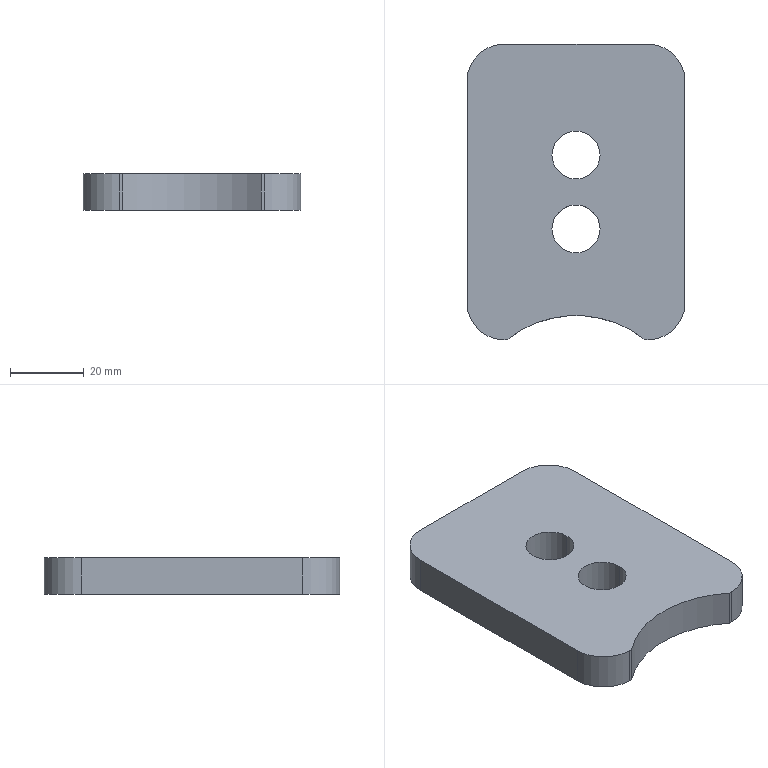Component | SolidWorks | 12ASlidingPlateWheelCover-3 | 1 solid | 16 faces | box 59 x 80 x 10 mm | volume 42016 mm3 | cylinder 9 | plane 7 | commonest cylinder face diameters 13 x4 20 x4 60 x1 | material Q235
build123d program:
from build123d import *

# Parameters (mm, degrees)
SKETCH1_W           = 59
SKETCH1_H           = 80
SKETCH1_R           = 6.5
BOSS_EXTRUDE1_DEPTH = 10
FILLET1_R           = 10
SKETCH2_R           = 30
CUT_EXTRUDE1_DEPTH  = 51.698


with BuildPart() as part:
    # Sketch1 → Boss-Extrude1 (new body)
    with BuildSketch(Plane.XY):
        Rectangle(SKETCH1_W, SKETCH1_H)
        with Locations((0, 10)):
            Circle(SKETCH1_R, mode=Mode.SUBTRACT)
        with Locations((0, -10)):
            Circle(SKETCH1_R, mode=Mode.SUBTRACT)
    extrude(amount=BOSS_EXTRUDE1_DEPTH)

    # Fillet1
    fillet1_edges = [part.edges().sort_by_distance(p)[0] for p in [
        (-29.5, 40, 5),
        (29.5, 40, 5),
        (29.5, -40, 5),
        (-29.5, -40, 5),
    ]]
    fillet(fillet1_edges, radius=FILLET1_R)

    # Sketch2 → Cut-Extrude1 (cut, through all)
    with BuildSketch(Plane.XY.offset(10)):
        with Locations((0, -63.457)):
            Circle(SKETCH2_R)
    extrude(amount=-CUT_EXTRUDE1_DEPTH, mode=Mode.SUBTRACT)


solid = part.part

# Placed as in the assembly
solid = solid.moved(Location((346.598, 136.538, -24.25), (0, 0, 0)))
STEP:
#1=CARTESIAN_POINT('',(13.39,4.982,-0.561));
#2=VERTEX_POINT('',#1);
#3=CARTESIAN_POINT('',(13.902,4.982,-0.561));
#4=VERTEX_POINT('',#3);
#5=CARTESIAN_POINT('',(13.646,4.982,-0.561));
#6=DIRECTION('',(0.,0.,1.));
#7=DIRECTION('',(1.,0.,0.));
#8=AXIS2_PLACEMENT_3D('',#5,#6,#7);
#9=CIRCLE('',#8,0.2559);
#10=EDGE_CURVE('',#2,#4,#9,.T.);
#11=ORIENTED_EDGE('',*,*,#10,.T.);
#12=CARTESIAN_POINT('',(13.902,4.982,-0.9547));
#13=VERTEX_POINT('',#12);
#14=CARTESIAN_POINT('',(13.902,4.982,-0.561));
#15=DIRECTION('',(0.,0.,-1.));
#16=VECTOR('',#15,39.37);
#17=LINE('',#14,#16);
#18=EDGE_CURVE('',#4,#13,#17,.T.);
#19=ORIENTED_EDGE('',*,*,#18,.T.);
#20=CARTESIAN_POINT('',(13.39,4.982,-0.9547));
#21=VERTEX_POINT('',#20);
#22=CARTESIAN_POINT('',(13.646,4.982,-0.9547));
#23=DIRECTION('',(0.,0.,1.));
#24=DIRECTION('',(1.,0.,0.));
#25=AXIS2_PLACEMENT_3D('',#22,#23,#24);
#26=CIRCLE('',#25,0.2559);
#27=EDGE_CURVE('',#21,#13,#26,.T.);
#28=ORIENTED_EDGE('',*,*,#27,.F.);
#29=CARTESIAN_POINT('',(13.39,4.982,-0.561));
#30=DIRECTION('',(0.,0.,-1.));
#31=VECTOR('',#30,39.37);
#32=LINE('',#29,#31);
#33=EDGE_CURVE('',#2,#21,#32,.T.);
#34=ORIENTED_EDGE('',*,*,#33,.F.);
#35=EDGE_LOOP('',(#11,#19,#28,#34));
#36=FACE_OUTER_BOUND('',#35,.T.);
#37=CARTESIAN_POINT('',(13.646,4.982,-0.561));
#38=DIRECTION('',(0.,0.,-1.));
#39=DIRECTION('',(-1.,0.,0.));
#40=AXIS2_PLACEMENT_3D('',#37,#38,#39);
#41=CYLINDRICAL_SURFACE('',#40,0.2559);
#42=ADVANCED_FACE('',(#36),#41,.F.);
#43=CARTESIAN_POINT('',(13.39,5.769,-0.561));
#44=VERTEX_POINT('',#43);
#45=CARTESIAN_POINT('',(13.902,5.769,-0.561));
#46=VERTEX_POINT('',#45);
#47=CARTESIAN_POINT('',(13.646,5.769,-0.561));
#48=DIRECTION('',(0.,0.,1.));
#49=DIRECTION('',(1.,0.,0.));
#50=AXIS2_PLACEMENT_3D('',#47,#48,#49);
#51=CIRCLE('',#50,0.2559);
#52=EDGE_CURVE('',#44,#46,#51,.T.);
#53=ORIENTED_EDGE('',*,*,#52,.T.);
#54=CARTESIAN_POINT('',(13.902,5.769,-0.9547));
#55=VERTEX_POINT('',#54);
#56=CARTESIAN_POINT('',(13.902,5.769,-0.561));
#57=DIRECTION('',(0.,0.,-1.));
#58=VECTOR('',#57,39.37);
#59=LINE('',#56,#58);
#60=EDGE_CURVE('',#46,#55,#59,.T.);
#61=ORIENTED_EDGE('',*,*,#60,.T.);
#62=CARTESIAN_POINT('',(13.39,5.769,-0.9547));
#63=VERTEX_POINT('',#62);
#64=CARTESIAN_POINT('',(13.646,5.769,-0.9547));
#65=DIRECTION('',(0.,0.,1.));
#66=DIRECTION('',(1.,0.,0.));
#67=AXIS2_PLACEMENT_3D('',#64,#65,#66);
#68=CIRCLE('',#67,0.2559);
#69=EDGE_CURVE('',#63,#55,#68,.T.);
#70=ORIENTED_EDGE('',*,*,#69,.F.);
#71=CARTESIAN_POINT('',(13.39,5.769,-0.561));
#72=DIRECTION('',(0.,0.,-1.));
#73=VECTOR('',#72,39.37);
#74=LINE('',#71,#73);
#75=EDGE_CURVE('',#44,#63,#74,.T.);
#76=ORIENTED_EDGE('',*,*,#75,.F.);
#77=EDGE_LOOP('',(#53,#61,#70,#76));
#78=FACE_OUTER_BOUND('',#77,.T.);
#79=CARTESIAN_POINT('',(13.646,5.769,-0.561));
#80=DIRECTION('',(0.,0.,-1.));
#81=DIRECTION('',(-1.,0.,0.));
#82=AXIS2_PLACEMENT_3D('',#79,#80,#81);
#83=CYLINDRICAL_SURFACE('',#82,0.2559);
#84=ADVANCED_FACE('',(#78),#83,.F.);
#85=CARTESIAN_POINT('',(12.878,3.801,-0.9547));
#86=VERTEX_POINT('',#85);
#87=CARTESIAN_POINT('',(12.909,3.801,-0.9547));
#88=VERTEX_POINT('',#87);
#89=CARTESIAN_POINT('',(12.484,3.801,-0.9547));
#90=DIRECTION('',(1.,0.,0.));
#91=VECTOR('',#90,39.37);
#92=LINE('',#89,#91);
#93=EDGE_CURVE('',#86,#88,#92,.T.);
#94=ORIENTED_EDGE('',*,*,#93,.T.);
#95=CARTESIAN_POINT('',(12.909,3.801,-0.561));
#96=VERTEX_POINT('',#95);
#97=CARTESIAN_POINT('',(12.909,3.801,-0.9547));
#98=DIRECTION('',(0.,0.,1.));
#99=VECTOR('',#98,39.37);
#100=LINE('',#97,#99);
#101=EDGE_CURVE('',#88,#96,#100,.T.);
#102=ORIENTED_EDGE('',*,*,#101,.T.);
#103=CARTESIAN_POINT('',(12.878,3.801,-0.561));
#104=VERTEX_POINT('',#103);
#105=CARTESIAN_POINT('',(12.484,3.801,-0.561));
#106=DIRECTION('',(1.,0.,0.));
#107=VECTOR('',#106,39.37);
#108=LINE('',#105,#107);
#109=EDGE_CURVE('',#104,#96,#108,.T.);
#110=ORIENTED_EDGE('',*,*,#109,.F.);
#111=CARTESIAN_POINT('',(12.878,3.801,-0.561));
#112=DIRECTION('',(0.,0.,-1.));
#113=VECTOR('',#112,39.37);
#114=LINE('',#111,#113);
#115=EDGE_CURVE('',#104,#86,#114,.T.);
#116=ORIENTED_EDGE('',*,*,#115,.T.);
#117=EDGE_LOOP('',(#94,#102,#110,#116));
#118=FACE_OUTER_BOUND('',#117,.T.);
#119=CARTESIAN_POINT('',(12.484,3.801,-0.561));
#120=DIRECTION('',(0.,1.,0.));
#121=DIRECTION('',(0.,0.,1.));
#122=AXIS2_PLACEMENT_3D('',#119,#120,#121);
#123=PLANE('',#122);
#124=ADVANCED_FACE('',(#118),#123,.F.);
#125=CARTESIAN_POINT('',(14.382,3.801,-0.561));
#126=VERTEX_POINT('',#125);
#127=CARTESIAN_POINT('',(13.646,2.877,-0.561));
#128=DIRECTION('',(0.,0.,1.));
#129=DIRECTION('',(1.,0.,0.));
#130=AXIS2_PLACEMENT_3D('',#127,#128,#129);
#131=CIRCLE('',#130,1.181);
#132=EDGE_CURVE('',#126,#96,#131,.T.);
#133=ORIENTED_EDGE('',*,*,#132,.F.);
#134=CARTESIAN_POINT('',(14.413,3.801,-0.561));
#135=VERTEX_POINT('',#134);
#136=CARTESIAN_POINT('',(12.484,3.801,-0.561));
#137=DIRECTION('',(1.,0.,0.));
#138=VECTOR('',#137,39.37);
#139=LINE('',#136,#138);
#140=EDGE_CURVE('',#126,#135,#139,.T.);
#141=ORIENTED_EDGE('',*,*,#140,.T.);
#142=CARTESIAN_POINT('',(14.807,4.194,-0.561));
#143=VERTEX_POINT('',#142);
#144=CARTESIAN_POINT('',(14.413,4.194,-0.561));
#145=DIRECTION('',(0.,0.,1.));
#146=DIRECTION('',(1.,0.,0.));
#147=AXIS2_PLACEMENT_3D('',#144,#145,#146);
#148=CIRCLE('',#147,0.3937);
#149=EDGE_CURVE('',#135,#143,#148,.T.);
#150=ORIENTED_EDGE('',*,*,#149,.T.);
#151=CARTESIAN_POINT('',(14.807,6.557,-0.561));
#152=VERTEX_POINT('',#151);
#153=CARTESIAN_POINT('',(14.807,6.95,-0.561));
#154=DIRECTION('',(-0.,1.,0.));
#155=VECTOR('',#154,39.37);
#156=LINE('',#153,#155);
#157=EDGE_CURVE('',#143,#152,#156,.T.);
#158=ORIENTED_EDGE('',*,*,#157,.T.);
#159=CARTESIAN_POINT('',(14.413,6.95,-0.561));
#160=VERTEX_POINT('',#159);
#161=CARTESIAN_POINT('',(14.413,6.557,-0.561));
#162=DIRECTION('',(0.,0.,1.));
#163=DIRECTION('',(1.,0.,0.));
#164=AXIS2_PLACEMENT_3D('',#161,#162,#163);
#165=CIRCLE('',#164,0.3937);
#166=EDGE_CURVE('',#152,#160,#165,.T.);
#167=ORIENTED_EDGE('',*,*,#166,.T.);
#168=CARTESIAN_POINT('',(12.878,6.95,-0.561));
#169=VERTEX_POINT('',#168);
#170=CARTESIAN_POINT('',(12.484,6.95,-0.561));
#171=DIRECTION('',(-1.,-0.,0.));
#172=VECTOR('',#171,39.37);
#173=LINE('',#170,#172);
#174=EDGE_CURVE('',#160,#169,#173,.T.);
#175=ORIENTED_EDGE('',*,*,#174,.T.);
#176=CARTESIAN_POINT('',(12.484,6.557,-0.561));
#177=VERTEX_POINT('',#176);
#178=CARTESIAN_POINT('',(12.878,6.557,-0.561));
#179=DIRECTION('',(0.,0.,1.));
#180=DIRECTION('',(1.,0.,0.));
#181=AXIS2_PLACEMENT_3D('',#178,#179,#180);
#182=CIRCLE('',#181,0.3937);
#183=EDGE_CURVE('',#169,#177,#182,.T.);
#184=ORIENTED_EDGE('',*,*,#183,.T.);
#185=CARTESIAN_POINT('',(12.484,4.194,-0.561));
#186=VERTEX_POINT('',#185);
#187=CARTESIAN_POINT('',(12.484,6.95,-0.561));
#188=DIRECTION('',(0.,-1.,0.));
#189=VECTOR('',#188,39.37);
#190=LINE('',#187,#189);
#191=EDGE_CURVE('',#177,#186,#190,.T.);
#192=ORIENTED_EDGE('',*,*,#191,.T.);
#193=CARTESIAN_POINT('',(12.878,4.194,-0.561));
#194=DIRECTION('',(0.,0.,1.));
#195=DIRECTION('',(1.,0.,0.));
#196=AXIS2_PLACEMENT_3D('',#193,#194,#195);
#197=CIRCLE('',#196,0.3937);
#198=EDGE_CURVE('',#186,#104,#197,.T.);
#199=ORIENTED_EDGE('',*,*,#198,.T.);
#200=ORIENTED_EDGE('',*,*,#109,.T.);
#201=EDGE_LOOP('',(#133,#141,#150,#158,#167,#175,#184,#192,#199,#200));
#202=FACE_OUTER_BOUND('',#201,.T.);
#203=ORIENTED_EDGE('',*,*,#52,.F.);
#204=CARTESIAN_POINT('',(13.646,5.769,-0.561));
#205=DIRECTION('',(0.,0.,1.));
#206=DIRECTION('',(1.,0.,0.));
#207=AXIS2_PLACEMENT_3D('',#204,#205,#206);
#208=CIRCLE('',#207,0.2559);
#209=EDGE_CURVE('',#46,#44,#208,.T.);
#210=ORIENTED_EDGE('',*,*,#209,.F.);
#211=EDGE_LOOP('',(#203,#210));
#212=FACE_BOUND('',#211,.T.);
#213=ORIENTED_EDGE('',*,*,#10,.F.);
#214=CARTESIAN_POINT('',(13.646,4.982,-0.561));
#215=DIRECTION('',(0.,0.,1.));
#216=DIRECTION('',(1.,0.,0.));
#217=AXIS2_PLACEMENT_3D('',#214,#215,#216);
#218=CIRCLE('',#217,0.2559);
#219=EDGE_CURVE('',#4,#2,#218,.T.);
#220=ORIENTED_EDGE('',*,*,#219,.F.);
#221=EDGE_LOOP('',(#213,#220));
#222=FACE_BOUND('',#221,.T.);
#223=CARTESIAN_POINT('',(13.646,5.376,-0.561));
#224=DIRECTION('',(0.,0.,1.));
#225=DIRECTION('',(1.,0.,0.));
#226=AXIS2_PLACEMENT_3D('',#223,#224,#225);
#227=PLANE('',#226);
#228=ADVANCED_FACE('',(#202,#212,#222),#227,.T.);
#229=CARTESIAN_POINT('',(14.382,3.801,-0.9547));
#230=VERTEX_POINT('',#229);
#231=CARTESIAN_POINT('',(14.413,3.801,-0.9547));
#232=VERTEX_POINT('',#231);
#233=CARTESIAN_POINT('',(12.484,3.801,-0.9547));
#234=DIRECTION('',(1.,0.,0.));
#235=VECTOR('',#234,39.37);
#236=LINE('',#233,#235);
#237=EDGE_CURVE('',#230,#232,#236,.T.);
#238=ORIENTED_EDGE('',*,*,#237,.F.);
#239=CARTESIAN_POINT('',(13.646,2.877,-0.9547));
#240=DIRECTION('',(0.,0.,1.));
#241=DIRECTION('',(1.,0.,0.));
#242=AXIS2_PLACEMENT_3D('',#239,#240,#241);
#243=CIRCLE('',#242,1.181);
#244=EDGE_CURVE('',#230,#88,#243,.T.);
#245=ORIENTED_EDGE('',*,*,#244,.T.);
#246=ORIENTED_EDGE('',*,*,#93,.F.);
#247=CARTESIAN_POINT('',(12.484,4.194,-0.9547));
#248=VERTEX_POINT('',#247);
#249=CARTESIAN_POINT('',(12.878,4.194,-0.9547));
#250=DIRECTION('',(0.,0.,-1.));
#251=DIRECTION('',(1.,0.,0.));
#252=AXIS2_PLACEMENT_3D('',#249,#250,#251);
#253=CIRCLE('',#252,0.3937);
#254=EDGE_CURVE('',#86,#248,#253,.T.);
#255=ORIENTED_EDGE('',*,*,#254,.T.);
#256=CARTESIAN_POINT('',(12.484,6.557,-0.9547));
#257=VERTEX_POINT('',#256);
#258=CARTESIAN_POINT('',(12.484,6.95,-0.9547));
#259=DIRECTION('',(0.,-1.,0.));
#260=VECTOR('',#259,39.37);
#261=LINE('',#258,#260);
#262=EDGE_CURVE('',#257,#248,#261,.T.);
#263=ORIENTED_EDGE('',*,*,#262,.F.);
#264=CARTESIAN_POINT('',(12.878,6.95,-0.9547));
#265=VERTEX_POINT('',#264);
#266=CARTESIAN_POINT('',(12.878,6.557,-0.9547));
#267=DIRECTION('',(0.,0.,-1.));
#268=DIRECTION('',(1.,0.,0.));
#269=AXIS2_PLACEMENT_3D('',#266,#267,#268);
#270=CIRCLE('',#269,0.3937);
#271=EDGE_CURVE('',#257,#265,#270,.T.);
#272=ORIENTED_EDGE('',*,*,#271,.T.);
#273=CARTESIAN_POINT('',(14.413,6.95,-0.9547));
#274=VERTEX_POINT('',#273);
#275=CARTESIAN_POINT('',(12.484,6.95,-0.9547));
#276=DIRECTION('',(-1.,-0.,0.));
#277=VECTOR('',#276,39.37);
#278=LINE('',#275,#277);
#279=EDGE_CURVE('',#274,#265,#278,.T.);
#280=ORIENTED_EDGE('',*,*,#279,.F.);
#281=CARTESIAN_POINT('',(14.807,6.557,-0.9547));
#282=VERTEX_POINT('',#281);
#283=CARTESIAN_POINT('',(14.413,6.557,-0.9547));
#284=DIRECTION('',(0.,0.,-1.));
#285=DIRECTION('',(1.,0.,0.));
#286=AXIS2_PLACEMENT_3D('',#283,#284,#285);
#287=CIRCLE('',#286,0.3937);
#288=EDGE_CURVE('',#274,#282,#287,.T.);
#289=ORIENTED_EDGE('',*,*,#288,.T.);
#290=CARTESIAN_POINT('',(14.807,4.194,-0.9547));
#291=VERTEX_POINT('',#290);
#292=CARTESIAN_POINT('',(14.807,6.95,-0.9547));
#293=DIRECTION('',(-0.,1.,0.));
#294=VECTOR('',#293,39.37);
#295=LINE('',#292,#294);
#296=EDGE_CURVE('',#291,#282,#295,.T.);
#297=ORIENTED_EDGE('',*,*,#296,.F.);
#298=CARTESIAN_POINT('',(14.413,4.194,-0.9547));
#299=DIRECTION('',(0.,0.,-1.));
#300=DIRECTION('',(1.,0.,0.));
#301=AXIS2_PLACEMENT_3D('',#298,#299,#300);
#302=CIRCLE('',#301,0.3937);
#303=EDGE_CURVE('',#291,#232,#302,.T.);
#304=ORIENTED_EDGE('',*,*,#303,.T.);
#305=EDGE_LOOP('',(#238,#245,#246,#255,#263,#272,#280,#289,#297,#304));
#306=FACE_OUTER_BOUND('',#305,.T.);
#307=ORIENTED_EDGE('',*,*,#69,.T.);
#308=CARTESIAN_POINT('',(13.646,5.769,-0.9547));
#309=DIRECTION('',(0.,0.,1.));
#310=DIRECTION('',(1.,0.,0.));
#311=AXIS2_PLACEMENT_3D('',#308,#309,#310);
#312=CIRCLE('',#311,0.2559);
#313=EDGE_CURVE('',#55,#63,#312,.T.);
#314=ORIENTED_EDGE('',*,*,#313,.T.);
#315=EDGE_LOOP('',(#307,#314));
#316=FACE_BOUND('',#315,.T.);
#317=ORIENTED_EDGE('',*,*,#27,.T.);
#318=CARTESIAN_POINT('',(13.646,4.982,-0.9547));
#319=DIRECTION('',(0.,0.,1.));
#320=DIRECTION('',(1.,0.,0.));
#321=AXIS2_PLACEMENT_3D('',#318,#319,#320);
#322=CIRCLE('',#321,0.2559);
#323=EDGE_CURVE('',#13,#21,#322,.T.);
#324=ORIENTED_EDGE('',*,*,#323,.T.);
#325=EDGE_LOOP('',(#317,#324));
#326=FACE_BOUND('',#325,.T.);
#327=CARTESIAN_POINT('',(13.646,5.376,-0.9547));
#328=DIRECTION('',(0.,0.,1.));
#329=DIRECTION('',(1.,0.,0.));
#330=AXIS2_PLACEMENT_3D('',#327,#328,#329);
#331=PLANE('',#330);
#332=ADVANCED_FACE('',(#306,#316,#326),#331,.F.);
#333=ORIENTED_EDGE('',*,*,#262,.T.);
#334=CARTESIAN_POINT('',(12.484,4.194,-0.561));
#335=DIRECTION('',(0.,0.,1.));
#336=VECTOR('',#335,39.37);
#337=LINE('',#334,#336);
#338=EDGE_CURVE('',#248,#186,#337,.T.);
#339=ORIENTED_EDGE('',*,*,#338,.T.);
#340=ORIENTED_EDGE('',*,*,#191,.F.);
#341=CARTESIAN_POINT('',(12.484,6.557,-0.561));
#342=DIRECTION('',(0.,0.,-1.));
#343=VECTOR('',#342,39.37);
#344=LINE('',#341,#343);
#345=EDGE_CURVE('',#177,#257,#344,.T.);
#346=ORIENTED_EDGE('',*,*,#345,.T.);
#347=EDGE_LOOP('',(#333,#339,#340,#346));
#348=FACE_OUTER_BOUND('',#347,.T.);
#349=CARTESIAN_POINT('',(12.484,6.95,-0.561));
#350=DIRECTION('',(1.,0.,0.));
#351=DIRECTION('',(-0.,1.,0.));
#352=AXIS2_PLACEMENT_3D('',#349,#350,#351);
#353=PLANE('',#352);
#354=ADVANCED_FACE('',(#348),#353,.F.);
#355=ORIENTED_EDGE('',*,*,#140,.F.);
#356=CARTESIAN_POINT('',(14.382,3.801,-0.9547));
#357=DIRECTION('',(0.,0.,-1.));
#358=VECTOR('',#357,39.37);
#359=LINE('',#356,#358);
#360=EDGE_CURVE('',#126,#230,#359,.T.);
#361=ORIENTED_EDGE('',*,*,#360,.T.);
#362=ORIENTED_EDGE('',*,*,#237,.T.);
#363=CARTESIAN_POINT('',(14.413,3.801,-0.561));
#364=DIRECTION('',(0.,0.,1.));
#365=VECTOR('',#364,39.37);
#366=LINE('',#363,#365);
#367=EDGE_CURVE('',#232,#135,#366,.T.);
#368=ORIENTED_EDGE('',*,*,#367,.T.);
#369=EDGE_LOOP('',(#355,#361,#362,#368));
#370=FACE_OUTER_BOUND('',#369,.T.);
#371=CARTESIAN_POINT('',(12.484,3.801,-0.561));
#372=DIRECTION('',(0.,1.,0.));
#373=DIRECTION('',(0.,0.,1.));
#374=AXIS2_PLACEMENT_3D('',#371,#372,#373);
#375=PLANE('',#374);
#376=ADVANCED_FACE('',(#370),#375,.F.);
#377=ORIENTED_EDGE('',*,*,#157,.F.);
#378=CARTESIAN_POINT('',(14.807,4.194,-0.561));
#379=DIRECTION('',(0.,0.,-1.));
#380=VECTOR('',#379,39.37);
#381=LINE('',#378,#380);
#382=EDGE_CURVE('',#143,#291,#381,.T.);
#383=ORIENTED_EDGE('',*,*,#382,.T.);
#384=ORIENTED_EDGE('',*,*,#296,.T.);
#385=CARTESIAN_POINT('',(14.807,6.557,-0.561));
#386=DIRECTION('',(0.,0.,1.));
#387=VECTOR('',#386,39.37);
#388=LINE('',#385,#387);
#389=EDGE_CURVE('',#282,#152,#388,.T.);
#390=ORIENTED_EDGE('',*,*,#389,.T.);
#391=EDGE_LOOP('',(#377,#383,#384,#390));
#392=FACE_OUTER_BOUND('',#391,.T.);
#393=CARTESIAN_POINT('',(14.807,6.95,-0.561));
#394=DIRECTION('',(-1.,-0.,0.));
#395=DIRECTION('',(0.,-1.,0.));
#396=AXIS2_PLACEMENT_3D('',#393,#394,#395);
#397=PLANE('',#396);
#398=ADVANCED_FACE('',(#392),#397,.F.);
#399=ORIENTED_EDGE('',*,*,#279,.T.);
#400=CARTESIAN_POINT('',(12.878,6.95,-0.561));
#401=DIRECTION('',(0.,0.,1.));
#402=VECTOR('',#401,39.37);
#403=LINE('',#400,#402);
#404=EDGE_CURVE('',#265,#169,#403,.T.);
#405=ORIENTED_EDGE('',*,*,#404,.T.);
#406=ORIENTED_EDGE('',*,*,#174,.F.);
#407=CARTESIAN_POINT('',(14.413,6.95,-0.561));
#408=DIRECTION('',(0.,0.,-1.));
#409=VECTOR('',#408,39.37);
#410=LINE('',#407,#409);
#411=EDGE_CURVE('',#160,#274,#410,.T.);
#412=ORIENTED_EDGE('',*,*,#411,.T.);
#413=EDGE_LOOP('',(#399,#405,#406,#412));
#414=FACE_OUTER_BOUND('',#413,.T.);
#415=CARTESIAN_POINT('',(12.484,6.95,-0.561));
#416=DIRECTION('',(0.,-1.,0.));
#417=DIRECTION('',(1.,0.,0.));
#418=AXIS2_PLACEMENT_3D('',#415,#416,#417);
#419=PLANE('',#418);
#420=ADVANCED_FACE('',(#414),#419,.F.);
#421=ORIENTED_EDGE('',*,*,#60,.F.);
#422=ORIENTED_EDGE('',*,*,#209,.T.);
#423=ORIENTED_EDGE('',*,*,#75,.T.);
#424=ORIENTED_EDGE('',*,*,#313,.F.);
#425=EDGE_LOOP('',(#421,#422,#423,#424));
#426=FACE_OUTER_BOUND('',#425,.T.);
#427=CARTESIAN_POINT('',(13.646,5.769,-0.561));
#428=DIRECTION('',(0.,0.,-1.));
#429=DIRECTION('',(-1.,0.,0.));
#430=AXIS2_PLACEMENT_3D('',#427,#428,#429);
#431=CYLINDRICAL_SURFACE('',#430,0.2559);
#432=ADVANCED_FACE('',(#426),#431,.F.);
#433=ORIENTED_EDGE('',*,*,#18,.F.);
#434=ORIENTED_EDGE('',*,*,#219,.T.);
#435=ORIENTED_EDGE('',*,*,#33,.T.);
#436=ORIENTED_EDGE('',*,*,#323,.F.);
#437=EDGE_LOOP('',(#433,#434,#435,#436));
#438=FACE_OUTER_BOUND('',#437,.T.);
#439=CARTESIAN_POINT('',(13.646,4.982,-0.561));
#440=DIRECTION('',(0.,0.,-1.));
#441=DIRECTION('',(-1.,0.,0.));
#442=AXIS2_PLACEMENT_3D('',#439,#440,#441);
#443=CYLINDRICAL_SURFACE('',#442,0.2559);
#444=ADVANCED_FACE('',(#438),#443,.F.);
#445=ORIENTED_EDGE('',*,*,#198,.F.);
#446=ORIENTED_EDGE('',*,*,#338,.F.);
#447=ORIENTED_EDGE('',*,*,#254,.F.);
#448=ORIENTED_EDGE('',*,*,#115,.F.);
#449=EDGE_LOOP('',(#445,#446,#447,#448));
#450=FACE_OUTER_BOUND('',#449,.T.);
#451=CARTESIAN_POINT('',(12.878,4.194,-0.561));
#452=DIRECTION('',(0.,0.,-1.));
#453=DIRECTION('',(-1.,0.,0.));
#454=AXIS2_PLACEMENT_3D('',#451,#452,#453);
#455=CYLINDRICAL_SURFACE('',#454,0.3937);
#456=ADVANCED_FACE('',(#450),#455,.T.);
#457=ORIENTED_EDGE('',*,*,#149,.F.);
#458=ORIENTED_EDGE('',*,*,#367,.F.);
#459=ORIENTED_EDGE('',*,*,#303,.F.);
#460=ORIENTED_EDGE('',*,*,#382,.F.);
#461=EDGE_LOOP('',(#457,#458,#459,#460));
#462=FACE_OUTER_BOUND('',#461,.T.);
#463=CARTESIAN_POINT('',(14.413,4.194,-0.561));
#464=DIRECTION('',(0.,0.,-1.));
#465=DIRECTION('',(-1.,0.,0.));
#466=AXIS2_PLACEMENT_3D('',#463,#464,#465);
#467=CYLINDRICAL_SURFACE('',#466,0.3937);
#468=ADVANCED_FACE('',(#462),#467,.T.);
#469=ORIENTED_EDGE('',*,*,#183,.F.);
#470=ORIENTED_EDGE('',*,*,#404,.F.);
#471=ORIENTED_EDGE('',*,*,#271,.F.);
#472=ORIENTED_EDGE('',*,*,#345,.F.);
#473=EDGE_LOOP('',(#469,#470,#471,#472));
#474=FACE_OUTER_BOUND('',#473,.T.);
#475=CARTESIAN_POINT('',(12.878,6.557,-0.561));
#476=DIRECTION('',(0.,0.,-1.));
#477=DIRECTION('',(-1.,0.,0.));
#478=AXIS2_PLACEMENT_3D('',#475,#476,#477);
#479=CYLINDRICAL_SURFACE('',#478,0.3937);
#480=ADVANCED_FACE('',(#474),#479,.T.);
#481=ORIENTED_EDGE('',*,*,#166,.F.);
#482=ORIENTED_EDGE('',*,*,#389,.F.);
#483=ORIENTED_EDGE('',*,*,#288,.F.);
#484=ORIENTED_EDGE('',*,*,#411,.F.);
#485=EDGE_LOOP('',(#481,#482,#483,#484));
#486=FACE_OUTER_BOUND('',#485,.T.);
#487=CARTESIAN_POINT('',(14.413,6.557,-0.561));
#488=DIRECTION('',(0.,0.,-1.));
#489=DIRECTION('',(-1.,0.,0.));
#490=AXIS2_PLACEMENT_3D('',#487,#488,#489);
#491=CYLINDRICAL_SURFACE('',#490,0.3937);
#492=ADVANCED_FACE('',(#486),#491,.T.);
#493=ORIENTED_EDGE('',*,*,#244,.F.);
#494=ORIENTED_EDGE('',*,*,#360,.F.);
#495=ORIENTED_EDGE('',*,*,#132,.T.);
#496=ORIENTED_EDGE('',*,*,#101,.F.);
#497=EDGE_LOOP('',(#493,#494,#495,#496));
#498=FACE_OUTER_BOUND('',#497,.T.);
#499=CARTESIAN_POINT('',(13.646,2.877,-0.9547));
#500=DIRECTION('',(0.,0.,1.));
#501=DIRECTION('',(1.,0.,0.));
#502=AXIS2_PLACEMENT_3D('',#499,#500,#501);
#503=CYLINDRICAL_SURFACE('',#502,1.181);
#504=ADVANCED_FACE('',(#498),#503,.F.);
#505=CLOSED_SHELL('',(#42,#84,#124,#228,#332,#354,#376,#398,#420,#432,#444,#456,#468,#480,#492,#504));
#506=MANIFOLD_SOLID_BREP('',#505);
#507=CARTESIAN_POINT('',(0.,0.,0.));
#508=DIRECTION('',(0.,0.,1.));
#509=DIRECTION('',(1.,0.,0.));
#510=AXIS2_PLACEMENT_3D('',#507,#508,#509);
#511=(LENGTH_UNIT()NAMED_UNIT(*)SI_UNIT($,.METRE.));
#512=LENGTH_MEASURE_WITH_UNIT(LENGTH_MEASURE(0.0254),#511);
#513=DIMENSIONAL_EXPONENTS(1.,0.,0.,0.,0.,0.,0.);
#514=(CONVERSION_BASED_UNIT('',#512)LENGTH_UNIT()NAMED_UNIT(#513));
#515=UNCERTAINTY_MEASURE_WITH_UNIT(LENGTH_MEASURE(0.00001),#514,'','');
#516=(NAMED_UNIT(*)PLANE_ANGLE_UNIT()SI_UNIT($,.RADIAN.));
#517=(NAMED_UNIT(*)SI_UNIT($,.STERADIAN.)SOLID_ANGLE_UNIT());
#518=(GEOMETRIC_REPRESENTATION_CONTEXT(3)GLOBAL_UNCERTAINTY_ASSIGNED_CONTEXT((#515))GLOBAL_UNIT_ASSIGNED_CONTEXT((#514,#516,#517))REPRESENTATION_CONTEXT('',''));
#519=ADVANCED_BREP_SHAPE_REPRESENTATION('',(#506,#510),#518);
#520=COLOUR_RGB('',0.7922,0.8196,0.9333);
#521=FILL_AREA_STYLE_COLOUR('',#520);
#522=FILL_AREA_STYLE('',(#521));
#523=SURFACE_STYLE_FILL_AREA(#522);
#524=SURFACE_SIDE_STYLE('',(#523));
#525=SURFACE_STYLE_USAGE(.BOTH.,#524);
#526=PRESENTATION_STYLE_ASSIGNMENT((#525));
#527=STYLED_ITEM('',(#526),#506);
#528=PRESENTATION_LAYER_ASSIGNMENT('','',(#527));
#529=(LENGTH_UNIT()NAMED_UNIT(*)SI_UNIT($,.METRE.));
#530=LENGTH_MEASURE_WITH_UNIT(LENGTH_MEASURE(0.0254),#529);
#531=DIMENSIONAL_EXPONENTS(1.,0.,0.,0.,0.,0.,0.);
#532=(CONVERSION_BASED_UNIT('',#530)LENGTH_UNIT()NAMED_UNIT(#531));
#533=UNCERTAINTY_MEASURE_WITH_UNIT(LENGTH_MEASURE(0.00001),#532,'','');
#534=(NAMED_UNIT(*)PLANE_ANGLE_UNIT()SI_UNIT($,.RADIAN.));
#535=(NAMED_UNIT(*)SI_UNIT($,.STERADIAN.)SOLID_ANGLE_UNIT());
#536=(GEOMETRIC_REPRESENTATION_CONTEXT(3)GLOBAL_UNCERTAINTY_ASSIGNED_CONTEXT((#533))GLOBAL_UNIT_ASSIGNED_CONTEXT((#532,#534,#535))REPRESENTATION_CONTEXT('',''));
#537=MECHANICAL_DESIGN_GEOMETRIC_PRESENTATION_REPRESENTATION('',(#527),#536);